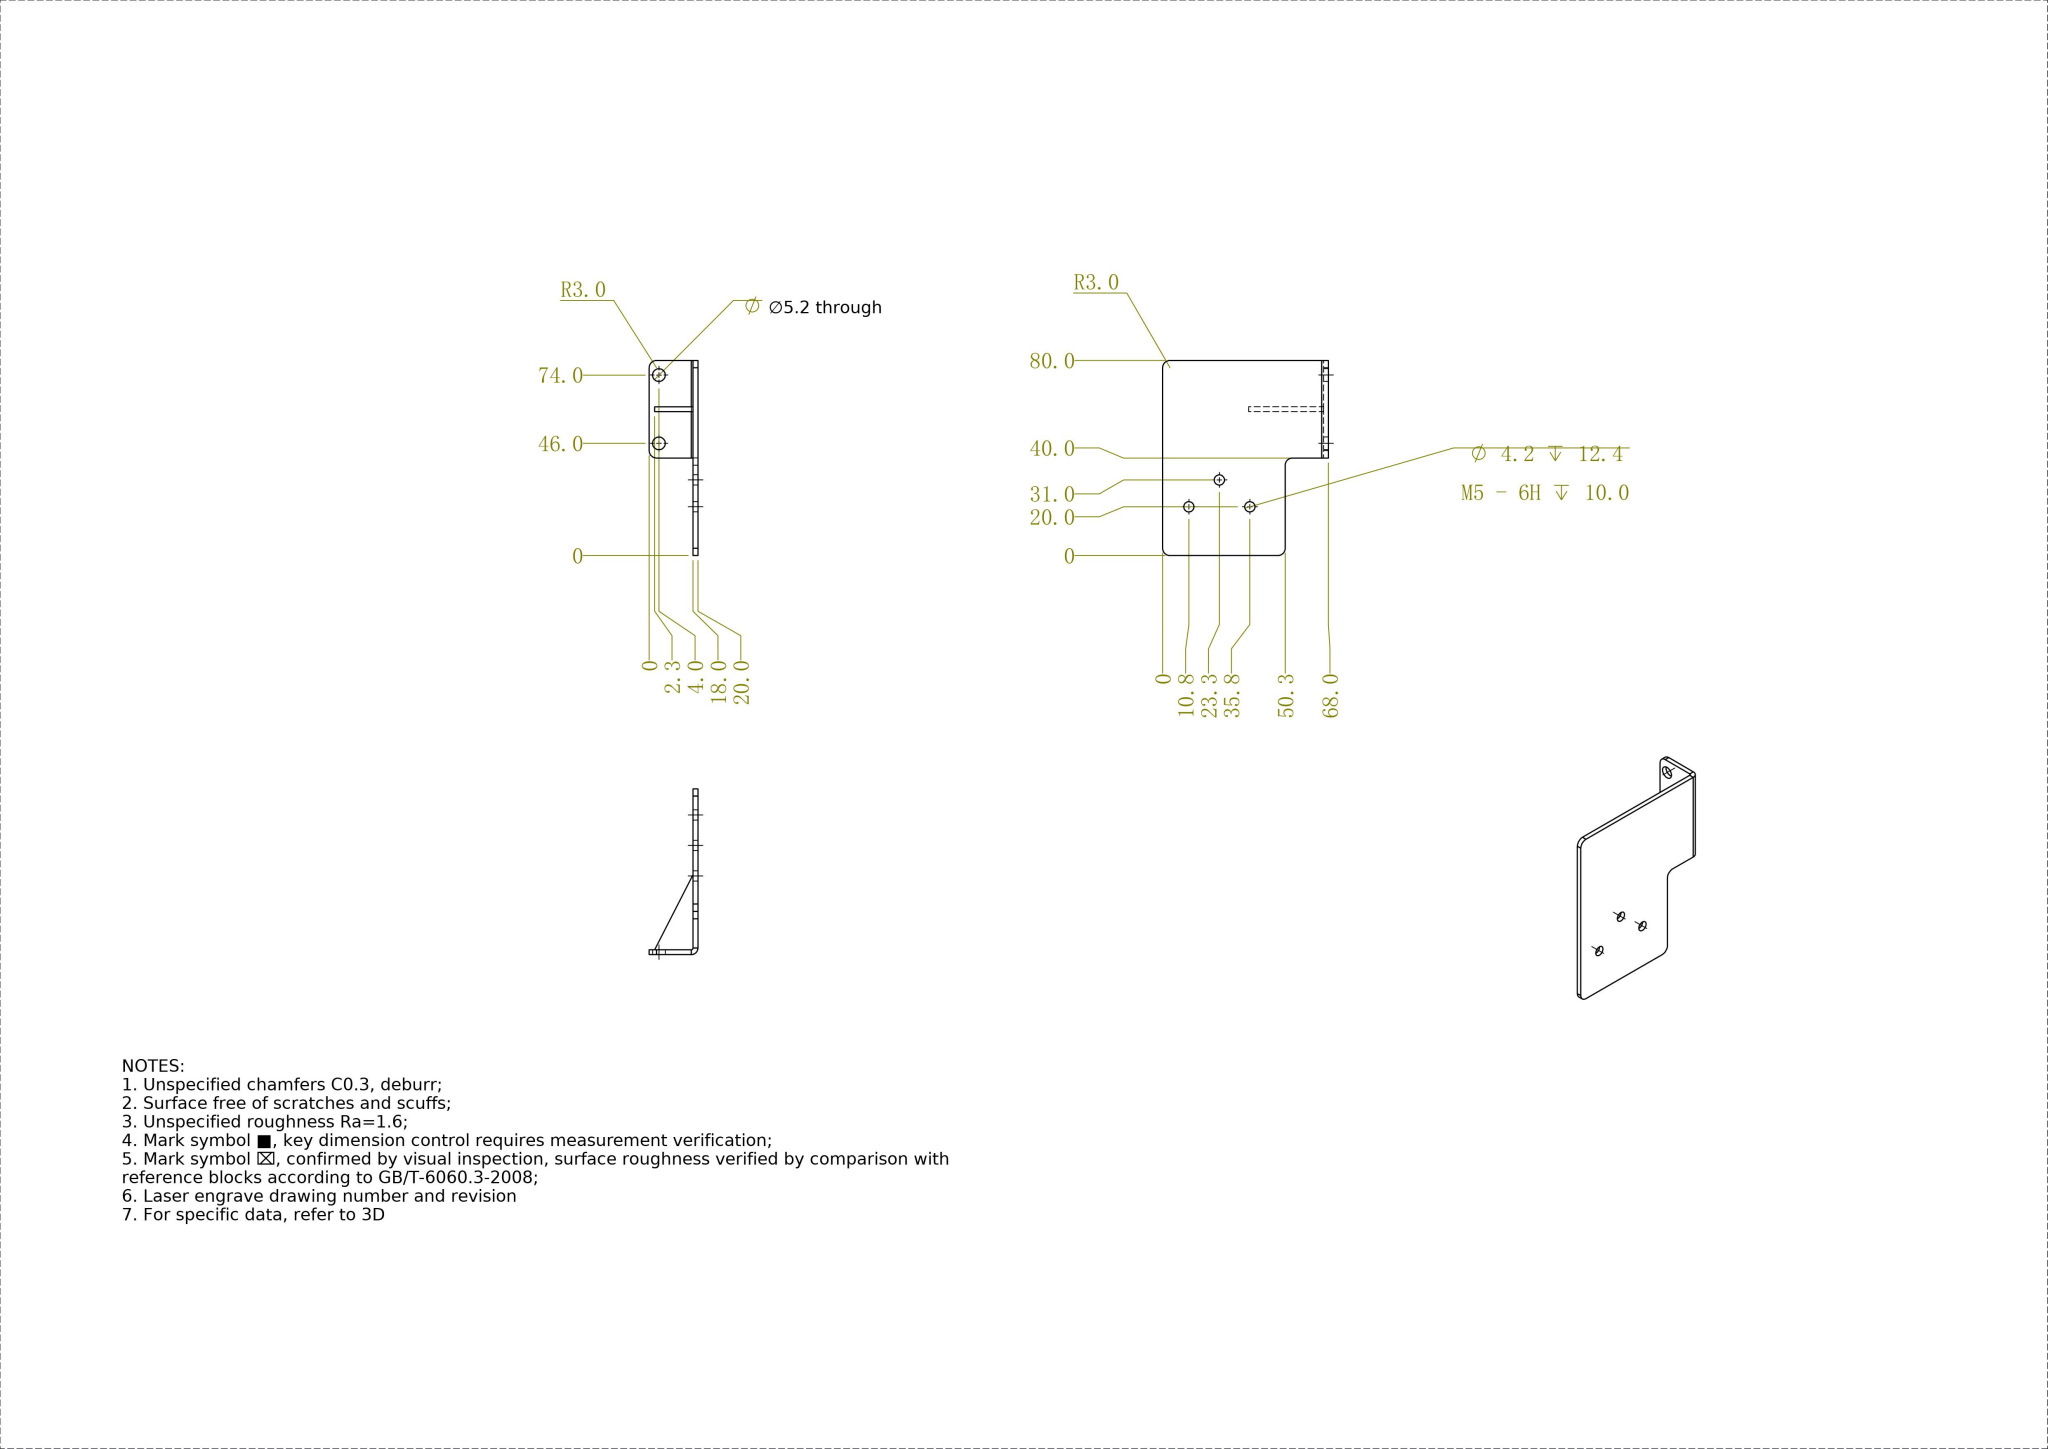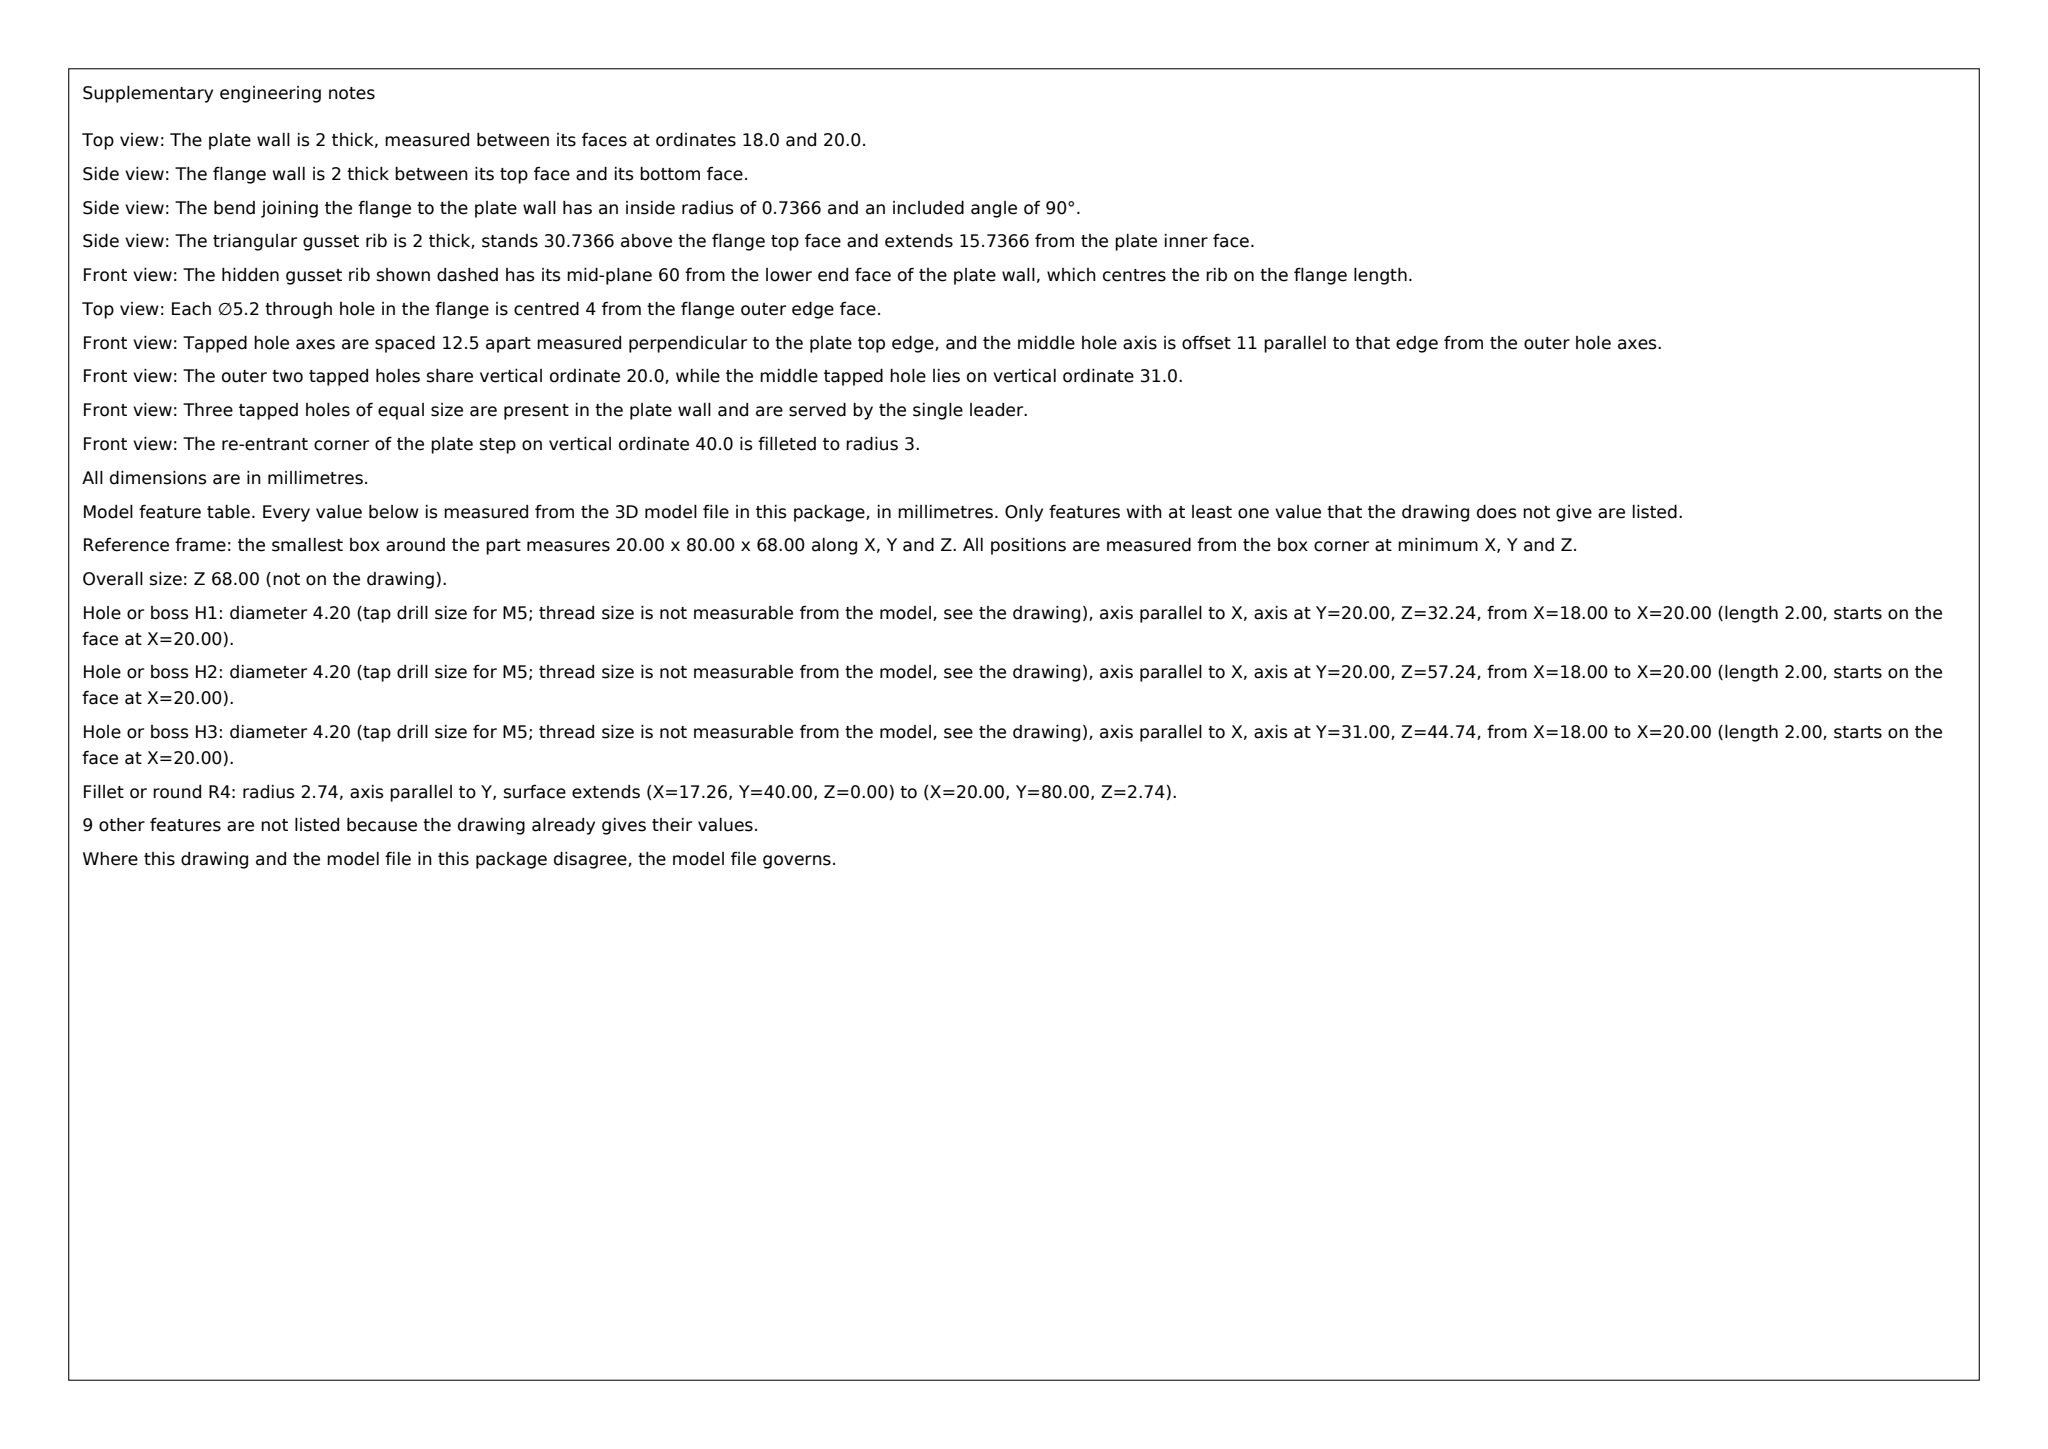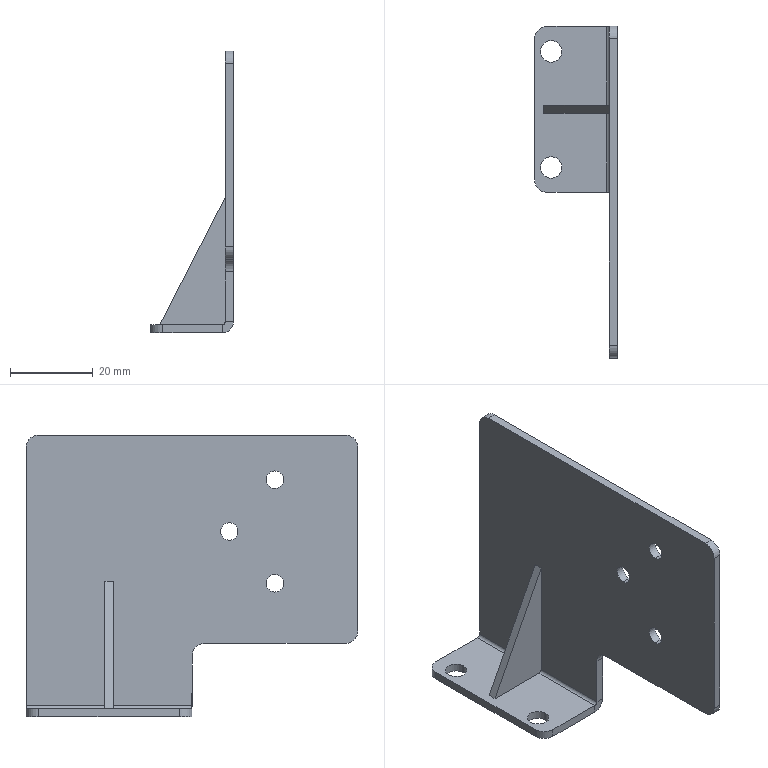Part | SolidWorks | mm | 1 solid | 36 faces | box 20 x 80 x 68 mm | volume 11141 mm3 | cylinder 19 | plane 17 | commonest cylinder face diameters 4.2 x6 6 x6 5.2 x4 1.473 x2 5.473 x1
Drawing notes:
BEND RELIEF SLOT 2.0 WIDE, Y59.0 TO Y61.0, THRU INNER R0.7 | from the solid: Planes y=59.0 and y=61.0 (2.0 apart); inner bend fillet Ø1.473 split into 2 segments of 19.0 over the 40.0 flange (19+2+19=40)
ALL CORNER RADII R3.0 TYP 6 PL, INCL INNER R AT 50.3/40.0 STEP | from the solid: Ø6.0 x 2.0 cyls: x-axis at (y3,z20.74),(y3,z65),(y37,z14.74 = inner corner of z=17.74/y=40 step),(y77,z65); z-axis at (x3,y43),(x3,y77)
3X Ø4.2 DP 12.4, M5-6H DP 10.0; 2X Ø5.2 THRU | from the solid: Ø4.2 x-axis holes at (y20,z32.24),(y20,z57.24),(y31,z44.74) = 35.8/10.8/23.3 from z=68; Ø5.2 z-axis holes at (x4,y46),(x4,y74)